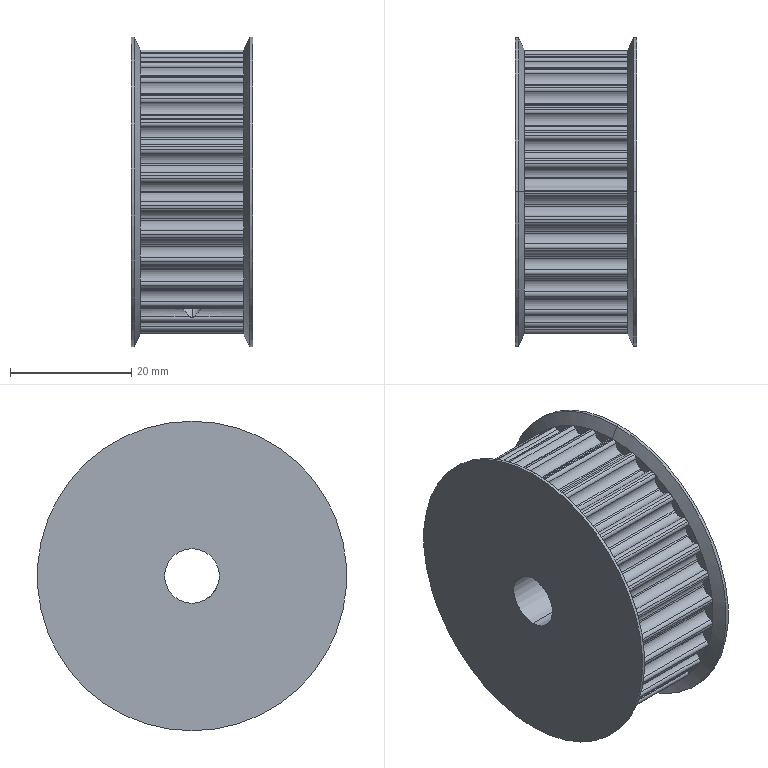Component | SolidWorks | 01000000A08029AS5MPulley2(Battery)122-1 | 1 solid | 263 faces | box 20 x 51 x 51 mm | volume 30941 mm3 | cylinder 165 | plane 94 | cone 4 | commonest cylinder face diameters 3 x64 1.1 x60 46.79 x31 3.3 x4 51 x4 9 x2
build123d program:
from build123d import *

# Parameters (mm, degrees)
EXTRUDE1_DEPTH    = 8.5
CIRPATTERN2_COUNT = 30
SKETCH5_W         = 1.65
SKETCH5_H         = 34.834
CIRPATTERN3_COUNT = 2
CIRPATTERN3_ANGLE = 120


with BuildPart() as part:
    # Sketch1 → Revolve1 (revolve)
    with BuildSketch(Plane.XY, mode=Mode.PRIVATE) as revolve1_sk:
        Polygon((-10, 4.5), (-10, 25.5), (-9.5, 25.5), (-8.5, 23.395), (8.5, 23.395), (9.5, 25.5), (10, 25.5), (10, 4.5), align=None)
    revolve(revolve1_sk.sketch.rotate(Axis((0, 0, 0), (1, 0, 0)), 90), axis=Axis((0, 0, 0), (1, 0, 0)))

    # Sketch2 → Extrude1 (cut, symmetric)
    with BuildSketch(Plane(origin=(0, 0, 0), x_dir=(0, 0, -1), z_dir=(1, 0, 0))):
        with BuildLine():
            Line((2.217, 23.29), (2.217, 38.448))
            Line((2.217, 38.448), (-2.217, 38.448))
            Line((-2.217, 38.448), (-2.217, 23.29))
            ThreePointArc((-2.217, 23.29), (-1.835, 23.182), (-1.625, 22.845))
            ThreePointArc((-1.625, 22.845), (-1.108, 21.97), (-0.1514, 21.625))
            Line((-0.1514, 21.625), (0.1514, 21.625))
            ThreePointArc((0.1514, 21.625), (1.108, 21.97), (1.625, 22.845))
            ThreePointArc((1.625, 22.845), (1.835, 23.182), (2.217, 23.29))
        make_face()
    extrude1 = extrude(amount=EXTRUDE1_DEPTH, both=True, mode=Mode.SUBTRACT)

    # CirPattern2: Extrude1 ×30 about axis
    cirpattern2_axis = Axis((0, 0, 0), (1, 0, 0))
    for i in range(1, CIRPATTERN2_COUNT):
        add(extrude1.rotate(cirpattern2_axis, i * 360 / CIRPATTERN2_COUNT), mode=Mode.SUBTRACT)

    # Sketch5 → M4 Tapped Hole1 (revolve, cut)
    with BuildSketch(Plane(origin=(0, 0, 0), x_dir=(0, 0, -1), z_dir=(1, 0, 0))):
        with Locations((0.825, 17.417)):
            Rectangle(SKETCH5_W, SKETCH5_H)
    m4_tapped_hole1 = revolve(axis=Axis((0, -6.35, 0), (0, 1, 0)), mode=Mode.SUBTRACT)

    # CirPattern3: M4 Tapped Hole1 ×2 about axis
    cirpattern3_axis = Axis((0, 0, 0), (-1, 0, 0))
    for i in range(1, CIRPATTERN3_COUNT):
        add(m4_tapped_hole1.rotate(cirpattern3_axis, i * CIRPATTERN3_ANGLE / (CIRPATTERN3_COUNT - 1)), mode=Mode.SUBTRACT)


solid = part.part

# Placed as in the assembly
solid = solid.moved(Location((-212.479, 448.741, 848.5), (0, 0, 0)))